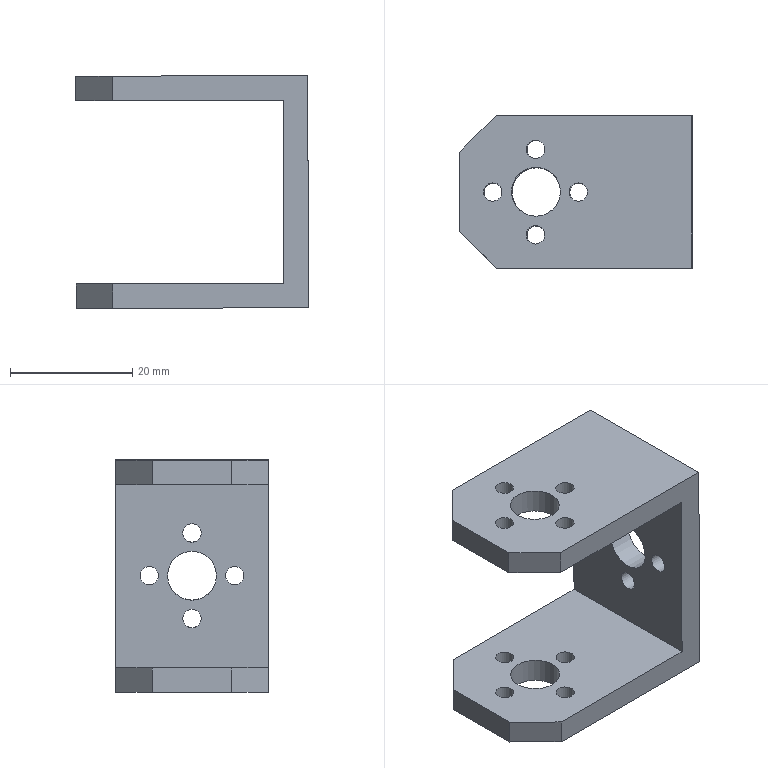Component | NX | U_SHAPE_2_3 | 1 solid | 29 faces | volume 9370 mm3 | cylinder 15 | plane 14 | commonest cylinder face diameters 3 x12 8 x3